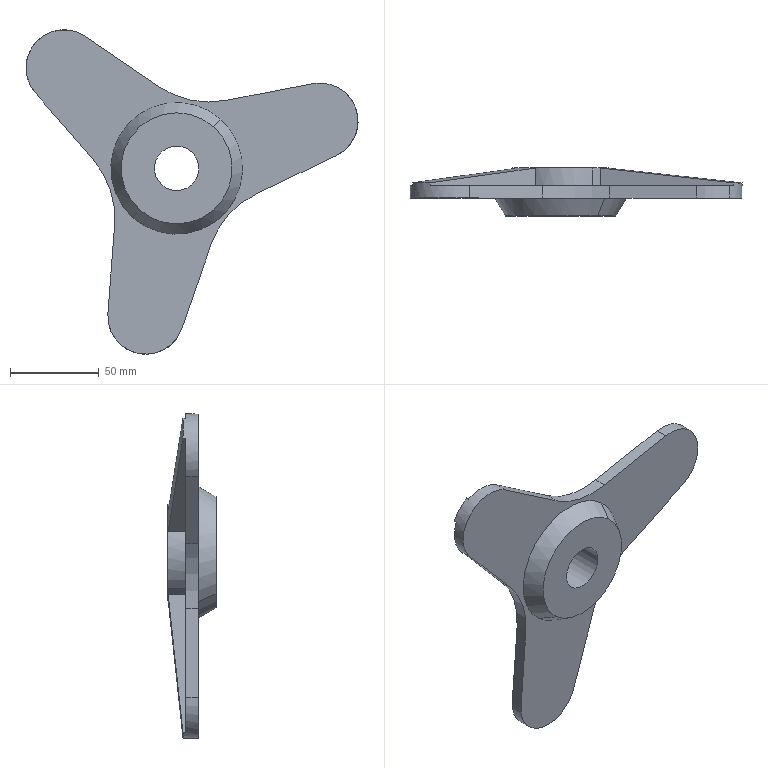Component | SolidWorks | Plug-2 | 1 solid | 34 faces | volume 167294 mm3 | plane 21 | cylinder 11 | cone 2 | commonest cylinder face diameters 42.868 x4 100 x3 25 x2 54 x2